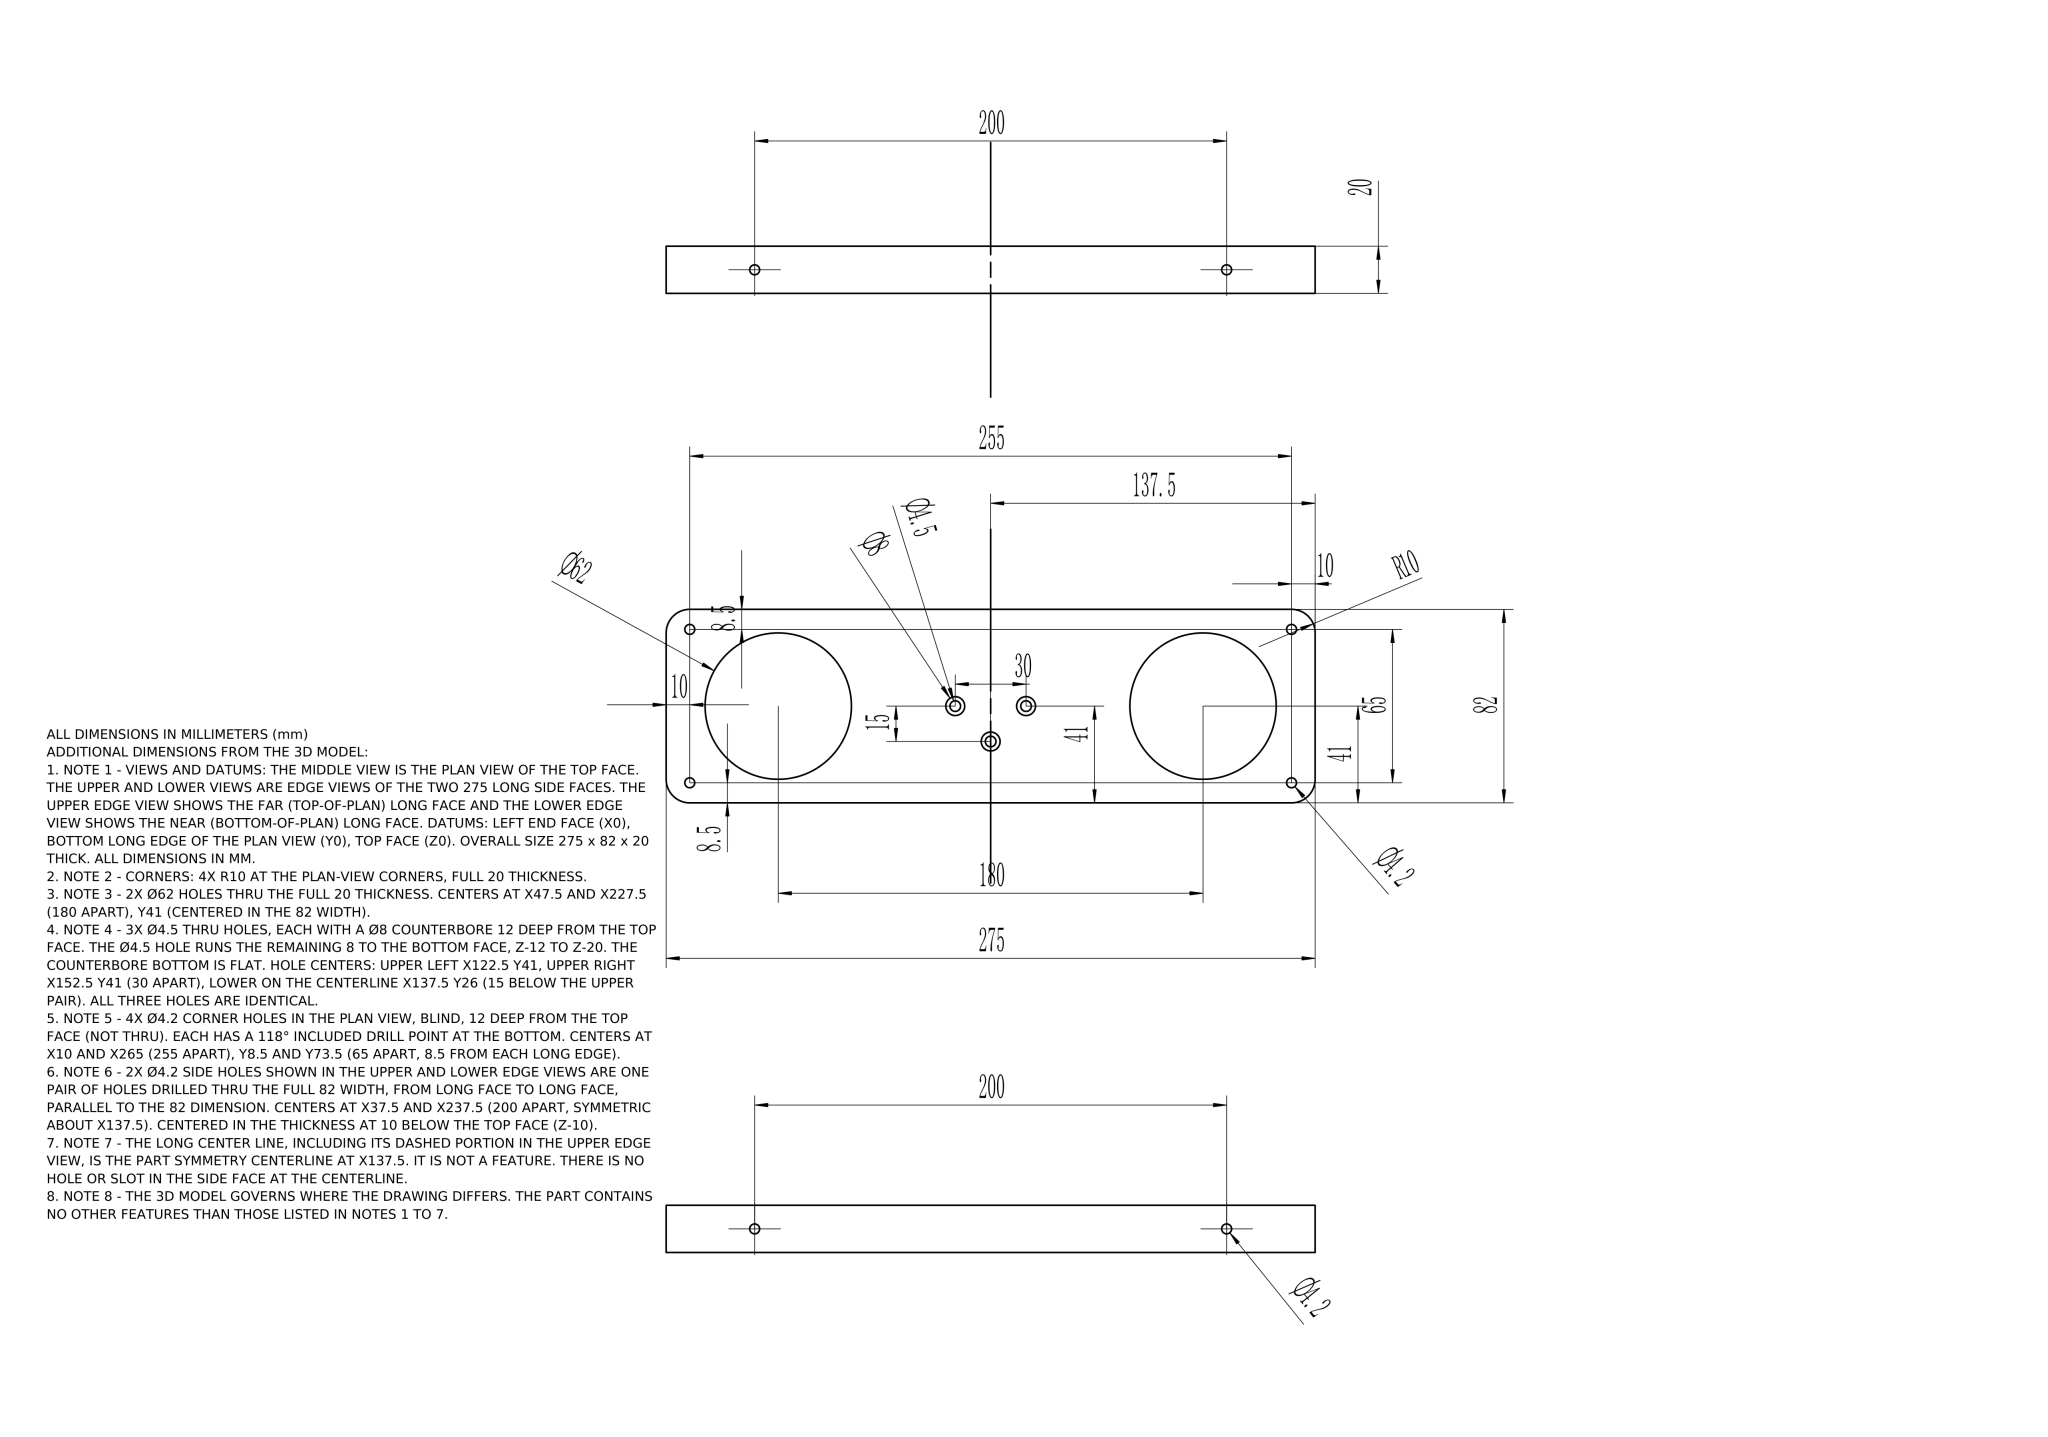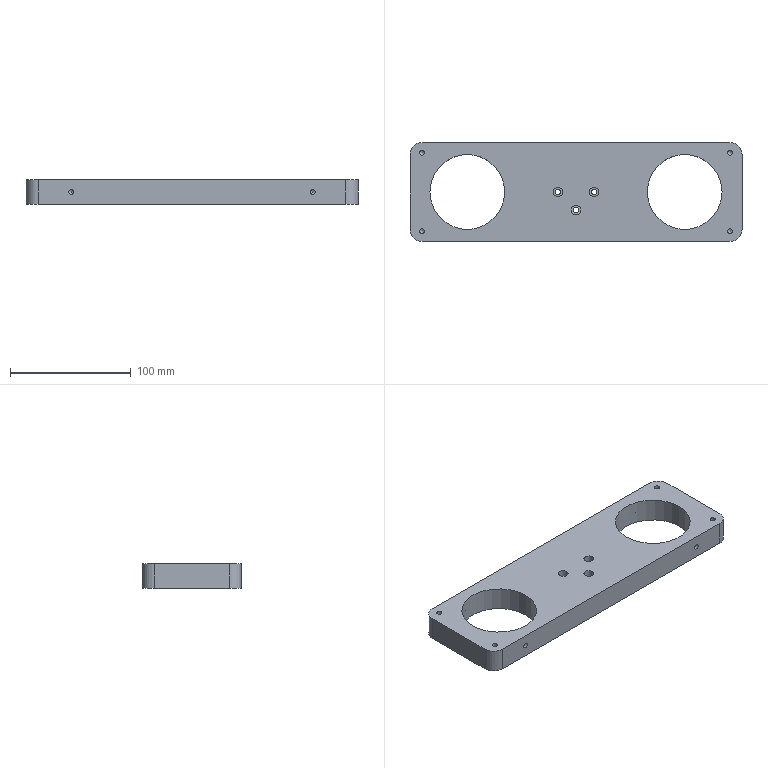Part | NX | mm | 1 solid | 37 faces | box 275 x 82 x 20 mm | volume 325063 mm3 | cylinder 20 | plane 9 | cone 8 | commonest cylinder face diameters 4.2 x8 20 x4 4.5 x3 8 x3 62 x2
STEP:
#1=CARTESIAN_POINT('',(0.,0.,0.));
#2=DIRECTION('',(0.,0.,1.));
#3=DIRECTION('',(1.,0.,0.));
#4=AXIS2_PLACEMENT_3D('',#1,#2,#3);
#5=(LENGTH_UNIT()NAMED_UNIT(*)SI_UNIT(.MILLI.,.METRE.));
#6=UNCERTAINTY_MEASURE_WITH_UNIT(LENGTH_MEASURE(0.00002),#5,'','');
#7=(NAMED_UNIT(*)PLANE_ANGLE_UNIT()SI_UNIT($,.RADIAN.));
#8=PLANE_ANGLE_MEASURE_WITH_UNIT(PLANE_ANGLE_MEASURE(0.01745),#7);
#9=DIMENSIONAL_EXPONENTS(0.,0.,0.,0.,0.,0.,0.);
#10=(CONVERSION_BASED_UNIT('',#8)NAMED_UNIT(#9)PLANE_ANGLE_UNIT());
#11=(NAMED_UNIT(*)SI_UNIT($,.STERADIAN.)SOLID_ANGLE_UNIT());
#12=(GEOMETRIC_REPRESENTATION_CONTEXT(3)GLOBAL_UNCERTAINTY_ASSIGNED_CONTEXT((#6))GLOBAL_UNIT_ASSIGNED_CONTEXT((#5,#10,#11))REPRESENTATION_CONTEXT('',''));
#13=SHAPE_REPRESENTATION('',(#4),#12);
#14=CARTESIAN_POINT('',(148.5,41.,0.));
#15=VERTEX_POINT('',#14);
#16=CARTESIAN_POINT('',(152.5,41.,0.));
#17=DIRECTION('',(0.,0.,-1.));
#18=DIRECTION('',(-1.,0.,0.));
#19=AXIS2_PLACEMENT_3D('',#16,#17,#18);
#20=CIRCLE('',#19,4.);
#21=EDGE_CURVE('',#15,#15,#20,.T.);
#22=ORIENTED_EDGE('',*,*,#21,.T.);
#23=EDGE_LOOP('',(#22));
#24=FACE_BOUND('',#23,.T.);
#25=CARTESIAN_POINT('',(133.5,26.,0.));
#26=VERTEX_POINT('',#25);
#27=CARTESIAN_POINT('',(137.5,26.,0.));
#28=DIRECTION('',(0.,0.,-1.));
#29=DIRECTION('',(-1.,0.,0.));
#30=AXIS2_PLACEMENT_3D('',#27,#28,#29);
#31=CIRCLE('',#30,4.);
#32=EDGE_CURVE('',#26,#26,#31,.T.);
#33=ORIENTED_EDGE('',*,*,#32,.T.);
#34=EDGE_LOOP('',(#33));
#35=FACE_BOUND('',#34,.T.);
#36=CARTESIAN_POINT('',(118.5,41.,0.));
#37=VERTEX_POINT('',#36);
#38=CARTESIAN_POINT('',(122.5,41.,0.));
#39=DIRECTION('',(0.,0.,-1.));
#40=DIRECTION('',(-1.,0.,0.));
#41=AXIS2_PLACEMENT_3D('',#38,#39,#40);
#42=CIRCLE('',#41,4.);
#43=EDGE_CURVE('',#37,#37,#42,.T.);
#44=ORIENTED_EDGE('',*,*,#43,.T.);
#45=EDGE_LOOP('',(#44));
#46=FACE_BOUND('',#45,.T.);
#47=CARTESIAN_POINT('',(262.9,73.5,0.));
#48=VERTEX_POINT('',#47);
#49=CARTESIAN_POINT('',(265.,73.5,0.));
#50=DIRECTION('',(0.,0.,-1.));
#51=DIRECTION('',(-1.,0.,0.));
#52=AXIS2_PLACEMENT_3D('',#49,#50,#51);
#53=CIRCLE('',#52,2.1);
#54=EDGE_CURVE('',#48,#48,#53,.T.);
#55=ORIENTED_EDGE('',*,*,#54,.T.);
#56=EDGE_LOOP('',(#55));
#57=FACE_BOUND('',#56,.T.);
#58=CARTESIAN_POINT('',(262.9,8.5,0.));
#59=VERTEX_POINT('',#58);
#60=CARTESIAN_POINT('',(265.,8.5,0.));
#61=DIRECTION('',(0.,0.,-1.));
#62=DIRECTION('',(-1.,0.,0.));
#63=AXIS2_PLACEMENT_3D('',#60,#61,#62);
#64=CIRCLE('',#63,2.1);
#65=EDGE_CURVE('',#59,#59,#64,.T.);
#66=ORIENTED_EDGE('',*,*,#65,.T.);
#67=EDGE_LOOP('',(#66));
#68=FACE_BOUND('',#67,.T.);
#69=CARTESIAN_POINT('',(7.9,73.5,0.));
#70=VERTEX_POINT('',#69);
#71=CARTESIAN_POINT('',(10.,73.5,0.));
#72=DIRECTION('',(0.,0.,-1.));
#73=DIRECTION('',(-1.,0.,0.));
#74=AXIS2_PLACEMENT_3D('',#71,#72,#73);
#75=CIRCLE('',#74,2.1);
#76=EDGE_CURVE('',#70,#70,#75,.T.);
#77=ORIENTED_EDGE('',*,*,#76,.T.);
#78=EDGE_LOOP('',(#77));
#79=FACE_BOUND('',#78,.T.);
#80=CARTESIAN_POINT('',(7.9,8.5,0.));
#81=VERTEX_POINT('',#80);
#82=CARTESIAN_POINT('',(10.,8.5,0.));
#83=DIRECTION('',(0.,0.,-1.));
#84=DIRECTION('',(-1.,0.,0.));
#85=AXIS2_PLACEMENT_3D('',#82,#83,#84);
#86=CIRCLE('',#85,2.1);
#87=EDGE_CURVE('',#81,#81,#86,.T.);
#88=ORIENTED_EDGE('',*,*,#87,.T.);
#89=EDGE_LOOP('',(#88));
#90=FACE_BOUND('',#89,.T.);
#91=CARTESIAN_POINT('',(196.5,41.,0.));
#92=VERTEX_POINT('',#91);
#93=CARTESIAN_POINT('',(227.5,41.,0.));
#94=DIRECTION('',(0.,0.,-1.));
#95=DIRECTION('',(-1.,0.,0.));
#96=AXIS2_PLACEMENT_3D('',#93,#94,#95);
#97=CIRCLE('',#96,31.);
#98=EDGE_CURVE('',#92,#92,#97,.T.);
#99=ORIENTED_EDGE('',*,*,#98,.T.);
#100=EDGE_LOOP('',(#99));
#101=FACE_BOUND('',#100,.T.);
#102=CARTESIAN_POINT('',(16.5,41.,0.));
#103=VERTEX_POINT('',#102);
#104=CARTESIAN_POINT('',(47.5,41.,0.));
#105=DIRECTION('',(0.,0.,-1.));
#106=DIRECTION('',(-1.,0.,0.));
#107=AXIS2_PLACEMENT_3D('',#104,#105,#106);
#108=CIRCLE('',#107,31.);
#109=EDGE_CURVE('',#103,#103,#108,.T.);
#110=ORIENTED_EDGE('',*,*,#109,.T.);
#111=EDGE_LOOP('',(#110));
#112=FACE_BOUND('',#111,.T.);
#113=CARTESIAN_POINT('',(275.,72.,0.));
#114=VERTEX_POINT('',#113);
#115=CARTESIAN_POINT('',(275.,10.,0.));
#116=VERTEX_POINT('',#115);
#117=CARTESIAN_POINT('',(275.,41.,0.));
#118=DIRECTION('',(0.,-1.,0.));
#119=VECTOR('',#118,1.);
#120=LINE('',#117,#119);
#121=EDGE_CURVE('',#114,#116,#120,.T.);
#122=ORIENTED_EDGE('',*,*,#121,.F.);
#123=CARTESIAN_POINT('',(265.,82.,0.));
#124=VERTEX_POINT('',#123);
#125=CARTESIAN_POINT('',(265.,72.,0.));
#126=DIRECTION('',(0.,0.,1.));
#127=DIRECTION('',(1.,0.,0.));
#128=AXIS2_PLACEMENT_3D('',#125,#126,#127);
#129=CIRCLE('',#128,10.);
#130=EDGE_CURVE('',#114,#124,#129,.T.);
#131=ORIENTED_EDGE('',*,*,#130,.T.);
#132=CARTESIAN_POINT('',(10.,82.,0.));
#133=VERTEX_POINT('',#132);
#134=CARTESIAN_POINT('',(137.5,82.,0.));
#135=DIRECTION('',(1.,0.,0.));
#136=VECTOR('',#135,1.);
#137=LINE('',#134,#136);
#138=EDGE_CURVE('',#133,#124,#137,.T.);
#139=ORIENTED_EDGE('',*,*,#138,.F.);
#140=CARTESIAN_POINT('',(0.,72.,0.));
#141=VERTEX_POINT('',#140);
#142=CARTESIAN_POINT('',(10.,72.,0.));
#143=DIRECTION('',(0.,0.,1.));
#144=DIRECTION('',(1.,0.,0.));
#145=AXIS2_PLACEMENT_3D('',#142,#143,#144);
#146=CIRCLE('',#145,10.);
#147=EDGE_CURVE('',#133,#141,#146,.T.);
#148=ORIENTED_EDGE('',*,*,#147,.T.);
#149=CARTESIAN_POINT('',(0.,10.,0.));
#150=VERTEX_POINT('',#149);
#151=CARTESIAN_POINT('',(0.,41.,0.));
#152=DIRECTION('',(0.,1.,0.));
#153=VECTOR('',#152,1.);
#154=LINE('',#151,#153);
#155=EDGE_CURVE('',#150,#141,#154,.T.);
#156=ORIENTED_EDGE('',*,*,#155,.F.);
#157=CARTESIAN_POINT('',(10.,0.,0.));
#158=VERTEX_POINT('',#157);
#159=CARTESIAN_POINT('',(10.,10.,0.));
#160=DIRECTION('',(0.,0.,1.));
#161=DIRECTION('',(1.,0.,0.));
#162=AXIS2_PLACEMENT_3D('',#159,#160,#161);
#163=CIRCLE('',#162,10.);
#164=EDGE_CURVE('',#150,#158,#163,.T.);
#165=ORIENTED_EDGE('',*,*,#164,.T.);
#166=CARTESIAN_POINT('',(265.,0.,0.));
#167=VERTEX_POINT('',#166);
#168=CARTESIAN_POINT('',(137.5,0.,0.));
#169=DIRECTION('',(-1.,0.,0.));
#170=VECTOR('',#169,1.);
#171=LINE('',#168,#170);
#172=EDGE_CURVE('',#167,#158,#171,.T.);
#173=ORIENTED_EDGE('',*,*,#172,.F.);
#174=CARTESIAN_POINT('',(265.,10.,0.));
#175=DIRECTION('',(0.,0.,1.));
#176=DIRECTION('',(1.,0.,0.));
#177=AXIS2_PLACEMENT_3D('',#174,#175,#176);
#178=CIRCLE('',#177,10.);
#179=EDGE_CURVE('',#167,#116,#178,.T.);
#180=ORIENTED_EDGE('',*,*,#179,.T.);
#181=EDGE_LOOP('',(#122,#131,#139,#148,#156,#165,#173,#180));
#182=FACE_BOUND('',#181,.T.);
#183=CARTESIAN_POINT('',(137.5,41.,0.));
#184=DIRECTION('',(0.,0.,1.));
#185=DIRECTION('',(1.,0.,0.));
#186=AXIS2_PLACEMENT_3D('',#183,#184,#185);
#187=PLANE('',#186);
#188=ADVANCED_FACE('',(#24,#35,#46,#57,#68,#79,#90,#101,#112,#182),#187,.T.);
#189=CARTESIAN_POINT('',(237.5,0.,-7.9));
#190=VERTEX_POINT('',#189);
#191=CARTESIAN_POINT('',(237.5,0.,-10.));
#192=DIRECTION('',(0.,1.,0.));
#193=DIRECTION('',(0.,0.,1.));
#194=AXIS2_PLACEMENT_3D('',#191,#192,#193);
#195=CIRCLE('',#194,2.1);
#196=EDGE_CURVE('',#190,#190,#195,.T.);
#197=ORIENTED_EDGE('',*,*,#196,.T.);
#198=EDGE_LOOP('',(#197));
#199=FACE_BOUND('',#198,.T.);
#200=CARTESIAN_POINT('',(37.5,0.,-7.9));
#201=VERTEX_POINT('',#200);
#202=CARTESIAN_POINT('',(37.5,0.,-10.));
#203=DIRECTION('',(0.,1.,0.));
#204=DIRECTION('',(0.,0.,1.));
#205=AXIS2_PLACEMENT_3D('',#202,#203,#204);
#206=CIRCLE('',#205,2.1);
#207=EDGE_CURVE('',#201,#201,#206,.T.);
#208=ORIENTED_EDGE('',*,*,#207,.T.);
#209=EDGE_LOOP('',(#208));
#210=FACE_BOUND('',#209,.T.);
#211=CARTESIAN_POINT('',(10.,0.,-20.));
#212=VERTEX_POINT('',#211);
#213=CARTESIAN_POINT('',(265.,0.,-20.));
#214=VERTEX_POINT('',#213);
#215=CARTESIAN_POINT('',(137.5,0.,-20.));
#216=DIRECTION('',(1.,0.,0.));
#217=VECTOR('',#216,1.);
#218=LINE('',#215,#217);
#219=EDGE_CURVE('',#212,#214,#218,.T.);
#220=ORIENTED_EDGE('',*,*,#219,.T.);
#221=CARTESIAN_POINT('',(265.,0.,-20.));
#222=DIRECTION('',(0.,0.,1.));
#223=VECTOR('',#222,1.);
#224=LINE('',#221,#223);
#225=EDGE_CURVE('',#214,#167,#224,.T.);
#226=ORIENTED_EDGE('',*,*,#225,.T.);
#227=ORIENTED_EDGE('',*,*,#172,.T.);
#228=CARTESIAN_POINT('',(10.,0.,-20.));
#229=DIRECTION('',(0.,0.,-1.));
#230=VECTOR('',#229,1.);
#231=LINE('',#228,#230);
#232=EDGE_CURVE('',#158,#212,#231,.T.);
#233=ORIENTED_EDGE('',*,*,#232,.T.);
#234=EDGE_LOOP('',(#220,#226,#227,#233));
#235=FACE_BOUND('',#234,.T.);
#236=CARTESIAN_POINT('',(137.5,0.,-20.));
#237=DIRECTION('',(0.,-1.,0.));
#238=DIRECTION('',(0.,0.,-1.));
#239=AXIS2_PLACEMENT_3D('',#236,#237,#238);
#240=PLANE('',#239);
#241=ADVANCED_FACE('',(#199,#210,#235),#240,.T.);
#242=ORIENTED_EDGE('',*,*,#155,.T.);
#243=CARTESIAN_POINT('',(0.,72.,-20.));
#244=VERTEX_POINT('',#243);
#245=CARTESIAN_POINT('',(0.,72.,-20.));
#246=DIRECTION('',(0.,0.,-1.));
#247=VECTOR('',#246,1.);
#248=LINE('',#245,#247);
#249=EDGE_CURVE('',#141,#244,#248,.T.);
#250=ORIENTED_EDGE('',*,*,#249,.T.);
#251=CARTESIAN_POINT('',(0.,10.,-20.));
#252=VERTEX_POINT('',#251);
#253=CARTESIAN_POINT('',(0.,41.,-20.));
#254=DIRECTION('',(0.,-1.,0.));
#255=VECTOR('',#254,1.);
#256=LINE('',#253,#255);
#257=EDGE_CURVE('',#244,#252,#256,.T.);
#258=ORIENTED_EDGE('',*,*,#257,.T.);
#259=CARTESIAN_POINT('',(0.,10.,-20.));
#260=DIRECTION('',(0.,0.,1.));
#261=VECTOR('',#260,1.);
#262=LINE('',#259,#261);
#263=EDGE_CURVE('',#252,#150,#262,.T.);
#264=ORIENTED_EDGE('',*,*,#263,.T.);
#265=EDGE_LOOP('',(#242,#250,#258,#264));
#266=FACE_OUTER_BOUND('',#265,.T.);
#267=CARTESIAN_POINT('',(0.,41.,-20.));
#268=DIRECTION('',(-1.,0.,0.));
#269=DIRECTION('',(0.,0.,1.));
#270=AXIS2_PLACEMENT_3D('',#267,#268,#269);
#271=PLANE('',#270);
#272=ADVANCED_FACE('',(#266),#271,.T.);
#273=CARTESIAN_POINT('',(237.5,82.,-12.1));
#274=VERTEX_POINT('',#273);
#275=CARTESIAN_POINT('',(237.5,82.,-10.));
#276=DIRECTION('',(0.,-1.,0.));
#277=DIRECTION('',(0.,0.,-1.));
#278=AXIS2_PLACEMENT_3D('',#275,#276,#277);
#279=CIRCLE('',#278,2.1);
#280=EDGE_CURVE('',#274,#274,#279,.T.);
#281=ORIENTED_EDGE('',*,*,#280,.T.);
#282=EDGE_LOOP('',(#281));
#283=FACE_BOUND('',#282,.T.);
#284=CARTESIAN_POINT('',(37.5,82.,-12.1));
#285=VERTEX_POINT('',#284);
#286=CARTESIAN_POINT('',(37.5,82.,-10.));
#287=DIRECTION('',(0.,-1.,0.));
#288=DIRECTION('',(0.,0.,-1.));
#289=AXIS2_PLACEMENT_3D('',#286,#287,#288);
#290=CIRCLE('',#289,2.1);
#291=EDGE_CURVE('',#285,#285,#290,.T.);
#292=ORIENTED_EDGE('',*,*,#291,.T.);
#293=EDGE_LOOP('',(#292));
#294=FACE_BOUND('',#293,.T.);
#295=ORIENTED_EDGE('',*,*,#138,.T.);
#296=CARTESIAN_POINT('',(265.,82.,-20.));
#297=VERTEX_POINT('',#296);
#298=CARTESIAN_POINT('',(265.,82.,-20.));
#299=DIRECTION('',(0.,0.,-1.));
#300=VECTOR('',#299,1.);
#301=LINE('',#298,#300);
#302=EDGE_CURVE('',#124,#297,#301,.T.);
#303=ORIENTED_EDGE('',*,*,#302,.T.);
#304=CARTESIAN_POINT('',(10.,82.,-20.));
#305=VERTEX_POINT('',#304);
#306=CARTESIAN_POINT('',(137.5,82.,-20.));
#307=DIRECTION('',(-1.,0.,0.));
#308=VECTOR('',#307,1.);
#309=LINE('',#306,#308);
#310=EDGE_CURVE('',#297,#305,#309,.T.);
#311=ORIENTED_EDGE('',*,*,#310,.T.);
#312=CARTESIAN_POINT('',(10.,82.,-20.));
#313=DIRECTION('',(0.,0.,1.));
#314=VECTOR('',#313,1.);
#315=LINE('',#312,#314);
#316=EDGE_CURVE('',#305,#133,#315,.T.);
#317=ORIENTED_EDGE('',*,*,#316,.T.);
#318=EDGE_LOOP('',(#295,#303,#311,#317));
#319=FACE_BOUND('',#318,.T.);
#320=CARTESIAN_POINT('',(137.5,82.,-20.));
#321=DIRECTION('',(0.,1.,0.));
#322=DIRECTION('',(0.,0.,1.));
#323=AXIS2_PLACEMENT_3D('',#320,#321,#322);
#324=PLANE('',#323);
#325=ADVANCED_FACE('',(#283,#294,#319),#324,.T.);
#326=CARTESIAN_POINT('',(150.25,41.,-20.));
#327=VERTEX_POINT('',#326);
#328=CARTESIAN_POINT('',(152.5,41.,-20.));
#329=DIRECTION('',(0.,0.,-1.));
#330=DIRECTION('',(-1.,0.,0.));
#331=AXIS2_PLACEMENT_3D('',#328,#329,#330);
#332=CIRCLE('',#331,2.25);
#333=EDGE_CURVE('',#327,#327,#332,.T.);
#334=ORIENTED_EDGE('',*,*,#333,.F.);
#335=EDGE_LOOP('',(#334));
#336=FACE_BOUND('',#335,.T.);
#337=CARTESIAN_POINT('',(135.25,26.,-20.));
#338=VERTEX_POINT('',#337);
#339=CARTESIAN_POINT('',(137.5,26.,-20.));
#340=DIRECTION('',(0.,0.,-1.));
#341=DIRECTION('',(-1.,0.,0.));
#342=AXIS2_PLACEMENT_3D('',#339,#340,#341);
#343=CIRCLE('',#342,2.25);
#344=EDGE_CURVE('',#338,#338,#343,.T.);
#345=ORIENTED_EDGE('',*,*,#344,.F.);
#346=EDGE_LOOP('',(#345));
#347=FACE_BOUND('',#346,.T.);
#348=CARTESIAN_POINT('',(120.25,41.,-20.));
#349=VERTEX_POINT('',#348);
#350=CARTESIAN_POINT('',(122.5,41.,-20.));
#351=DIRECTION('',(0.,0.,-1.));
#352=DIRECTION('',(-1.,0.,0.));
#353=AXIS2_PLACEMENT_3D('',#350,#351,#352);
#354=CIRCLE('',#353,2.25);
#355=EDGE_CURVE('',#349,#349,#354,.T.);
#356=ORIENTED_EDGE('',*,*,#355,.F.);
#357=EDGE_LOOP('',(#356));
#358=FACE_BOUND('',#357,.T.);
#359=CARTESIAN_POINT('',(196.5,41.,-20.));
#360=VERTEX_POINT('',#359);
#361=CARTESIAN_POINT('',(227.5,41.,-20.));
#362=DIRECTION('',(0.,0.,-1.));
#363=DIRECTION('',(-1.,0.,0.));
#364=AXIS2_PLACEMENT_3D('',#361,#362,#363);
#365=CIRCLE('',#364,31.);
#366=EDGE_CURVE('',#360,#360,#365,.T.);
#367=ORIENTED_EDGE('',*,*,#366,.F.);
#368=EDGE_LOOP('',(#367));
#369=FACE_BOUND('',#368,.T.);
#370=CARTESIAN_POINT('',(16.5,41.,-20.));
#371=VERTEX_POINT('',#370);
#372=CARTESIAN_POINT('',(47.5,41.,-20.));
#373=DIRECTION('',(0.,0.,-1.));
#374=DIRECTION('',(-1.,0.,0.));
#375=AXIS2_PLACEMENT_3D('',#372,#373,#374);
#376=CIRCLE('',#375,31.);
#377=EDGE_CURVE('',#371,#371,#376,.T.);
#378=ORIENTED_EDGE('',*,*,#377,.F.);
#379=EDGE_LOOP('',(#378));
#380=FACE_BOUND('',#379,.T.);
#381=ORIENTED_EDGE('',*,*,#310,.F.);
#382=CARTESIAN_POINT('',(275.,72.,-20.));
#383=VERTEX_POINT('',#382);
#384=CARTESIAN_POINT('',(265.,72.,-20.));
#385=DIRECTION('',(0.,0.,-1.));
#386=DIRECTION('',(-1.,0.,0.));
#387=AXIS2_PLACEMENT_3D('',#384,#385,#386);
#388=CIRCLE('',#387,10.);
#389=EDGE_CURVE('',#297,#383,#388,.T.);
#390=ORIENTED_EDGE('',*,*,#389,.T.);
#391=CARTESIAN_POINT('',(275.,10.,-20.));
#392=VERTEX_POINT('',#391);
#393=CARTESIAN_POINT('',(275.,41.,-20.));
#394=DIRECTION('',(0.,1.,0.));
#395=VECTOR('',#394,1.);
#396=LINE('',#393,#395);
#397=EDGE_CURVE('',#392,#383,#396,.T.);
#398=ORIENTED_EDGE('',*,*,#397,.F.);
#399=CARTESIAN_POINT('',(265.,10.,-20.));
#400=DIRECTION('',(0.,0.,-1.));
#401=DIRECTION('',(-1.,0.,0.));
#402=AXIS2_PLACEMENT_3D('',#399,#400,#401);
#403=CIRCLE('',#402,10.);
#404=EDGE_CURVE('',#392,#214,#403,.T.);
#405=ORIENTED_EDGE('',*,*,#404,.T.);
#406=ORIENTED_EDGE('',*,*,#219,.F.);
#407=CARTESIAN_POINT('',(10.,10.,-20.));
#408=DIRECTION('',(0.,0.,-1.));
#409=DIRECTION('',(-1.,0.,0.));
#410=AXIS2_PLACEMENT_3D('',#407,#408,#409);
#411=CIRCLE('',#410,10.);
#412=EDGE_CURVE('',#212,#252,#411,.T.);
#413=ORIENTED_EDGE('',*,*,#412,.T.);
#414=ORIENTED_EDGE('',*,*,#257,.F.);
#415=CARTESIAN_POINT('',(10.,72.,-20.));
#416=DIRECTION('',(0.,0.,-1.));
#417=DIRECTION('',(-1.,0.,0.));
#418=AXIS2_PLACEMENT_3D('',#415,#416,#417);
#419=CIRCLE('',#418,10.);
#420=EDGE_CURVE('',#244,#305,#419,.T.);
#421=ORIENTED_EDGE('',*,*,#420,.T.);
#422=EDGE_LOOP('',(#381,#390,#398,#405,#406,#413,#414,#421));
#423=FACE_BOUND('',#422,.T.);
#424=CARTESIAN_POINT('',(137.5,41.,-20.));
#425=DIRECTION('',(0.,0.,-1.));
#426=DIRECTION('',(-1.,0.,0.));
#427=AXIS2_PLACEMENT_3D('',#424,#425,#426);
#428=PLANE('',#427);
#429=ADVANCED_FACE('',(#336,#347,#358,#369,#380,#423),#428,.T.);
#430=ORIENTED_EDGE('',*,*,#397,.T.);
#431=CARTESIAN_POINT('',(275.,72.,-20.));
#432=DIRECTION('',(0.,0.,1.));
#433=VECTOR('',#432,1.);
#434=LINE('',#431,#433);
#435=EDGE_CURVE('',#383,#114,#434,.T.);
#436=ORIENTED_EDGE('',*,*,#435,.T.);
#437=ORIENTED_EDGE('',*,*,#121,.T.);
#438=CARTESIAN_POINT('',(275.,10.,-20.));
#439=DIRECTION('',(0.,0.,-1.));
#440=VECTOR('',#439,1.);
#441=LINE('',#438,#440);
#442=EDGE_CURVE('',#116,#392,#441,.T.);
#443=ORIENTED_EDGE('',*,*,#442,.T.);
#444=EDGE_LOOP('',(#430,#436,#437,#443));
#445=FACE_OUTER_BOUND('',#444,.T.);
#446=CARTESIAN_POINT('',(275.,41.,-20.));
#447=DIRECTION('',(1.,0.,0.));
#448=DIRECTION('',(0.,0.,-1.));
#449=AXIS2_PLACEMENT_3D('',#446,#447,#448);
#450=PLANE('',#449);
#451=ADVANCED_FACE('',(#445),#450,.T.);
#452=ORIENTED_EDGE('',*,*,#389,.F.);
#453=ORIENTED_EDGE('',*,*,#302,.F.);
#454=ORIENTED_EDGE('',*,*,#130,.F.);
#455=ORIENTED_EDGE('',*,*,#435,.F.);
#456=EDGE_LOOP('',(#452,#453,#454,#455));
#457=FACE_OUTER_BOUND('',#456,.T.);
#458=CARTESIAN_POINT('',(265.,72.,-20.));
#459=DIRECTION('',(0.,0.,1.));
#460=DIRECTION('',(1.,0.,0.));
#461=AXIS2_PLACEMENT_3D('',#458,#459,#460);
#462=CYLINDRICAL_SURFACE('',#461,10.);
#463=ADVANCED_FACE('',(#457),#462,.T.);
#464=ORIENTED_EDGE('',*,*,#404,.F.);
#465=ORIENTED_EDGE('',*,*,#442,.F.);
#466=ORIENTED_EDGE('',*,*,#179,.F.);
#467=ORIENTED_EDGE('',*,*,#225,.F.);
#468=EDGE_LOOP('',(#464,#465,#466,#467));
#469=FACE_OUTER_BOUND('',#468,.T.);
#470=CARTESIAN_POINT('',(265.,10.,-20.));
#471=DIRECTION('',(0.,0.,1.));
#472=DIRECTION('',(1.,0.,0.));
#473=AXIS2_PLACEMENT_3D('',#470,#471,#472);
#474=CYLINDRICAL_SURFACE('',#473,10.);
#475=ADVANCED_FACE('',(#469),#474,.T.);
#476=ORIENTED_EDGE('',*,*,#420,.F.);
#477=ORIENTED_EDGE('',*,*,#249,.F.);
#478=ORIENTED_EDGE('',*,*,#147,.F.);
#479=ORIENTED_EDGE('',*,*,#316,.F.);
#480=EDGE_LOOP('',(#476,#477,#478,#479));
#481=FACE_OUTER_BOUND('',#480,.T.);
#482=CARTESIAN_POINT('',(10.,72.,-20.));
#483=DIRECTION('',(0.,0.,1.));
#484=DIRECTION('',(1.,0.,0.));
#485=AXIS2_PLACEMENT_3D('',#482,#483,#484);
#486=CYLINDRICAL_SURFACE('',#485,10.);
#487=ADVANCED_FACE('',(#481),#486,.T.);
#488=ORIENTED_EDGE('',*,*,#412,.F.);
#489=ORIENTED_EDGE('',*,*,#232,.F.);
#490=ORIENTED_EDGE('',*,*,#164,.F.);
#491=ORIENTED_EDGE('',*,*,#263,.F.);
#492=EDGE_LOOP('',(#488,#489,#490,#491));
#493=FACE_OUTER_BOUND('',#492,.T.);
#494=CARTESIAN_POINT('',(10.,10.,-20.));
#495=DIRECTION('',(0.,0.,1.));
#496=DIRECTION('',(1.,0.,0.));
#497=AXIS2_PLACEMENT_3D('',#494,#495,#496);
#498=CYLINDRICAL_SURFACE('',#497,10.);
#499=ADVANCED_FACE('',(#493),#498,.T.);
#500=ORIENTED_EDGE('',*,*,#377,.T.);
#501=EDGE_LOOP('',(#500));
#502=FACE_BOUND('',#501,.T.);
#503=ORIENTED_EDGE('',*,*,#109,.F.);
#504=EDGE_LOOP('',(#503));
#505=FACE_BOUND('',#504,.T.);
#506=CARTESIAN_POINT('',(47.5,41.,0.));
#507=DIRECTION('',(0.,0.,-1.));
#508=DIRECTION('',(-1.,0.,0.));
#509=AXIS2_PLACEMENT_3D('',#506,#507,#508);
#510=CYLINDRICAL_SURFACE('',#509,31.);
#511=ADVANCED_FACE('',(#502,#505),#510,.F.);
#512=ORIENTED_EDGE('',*,*,#366,.T.);
#513=EDGE_LOOP('',(#512));
#514=FACE_BOUND('',#513,.T.);
#515=ORIENTED_EDGE('',*,*,#98,.F.);
#516=EDGE_LOOP('',(#515));
#517=FACE_BOUND('',#516,.T.);
#518=CARTESIAN_POINT('',(227.5,41.,0.));
#519=DIRECTION('',(0.,0.,-1.));
#520=DIRECTION('',(-1.,0.,0.));
#521=AXIS2_PLACEMENT_3D('',#518,#519,#520);
#522=CYLINDRICAL_SURFACE('',#521,31.);
#523=ADVANCED_FACE('',(#514,#517),#522,.F.);
#524=CARTESIAN_POINT('',(7.9,8.5,-12.));
#525=VERTEX_POINT('',#524);
#526=CARTESIAN_POINT('',(10.,8.5,-12.));
#527=DIRECTION('',(0.,0.,1.));
#528=DIRECTION('',(-1.,0.,0.));
#529=AXIS2_PLACEMENT_3D('',#526,#527,#528);
#530=CIRCLE('',#529,2.1);
#531=EDGE_CURVE('',#525,#525,#530,.T.);
#532=ORIENTED_EDGE('',*,*,#531,.T.);
#533=EDGE_LOOP('',(#532));
#534=FACE_BOUND('',#533,.T.);
#535=CARTESIAN_POINT('',(10.,8.5,-13.262));
#536=VERTEX_POINT('',#535);
#537=VERTEX_LOOP('',#536);
#538=FACE_BOUND('',#537,.T.);
#539=CARTESIAN_POINT('',(10.,8.5,-12.));
#540=DIRECTION('',(0.,0.,1.));
#541=DIRECTION('',(1.,0.,-0.));
#542=AXIS2_PLACEMENT_3D('',#539,#540,#541);
#543=CONICAL_SURFACE('',#542,2.1,59.);
#544=ADVANCED_FACE('',(#534,#538),#543,.F.);
#545=ORIENTED_EDGE('',*,*,#531,.F.);
#546=EDGE_LOOP('',(#545));
#547=FACE_BOUND('',#546,.T.);
#548=ORIENTED_EDGE('',*,*,#87,.F.);
#549=EDGE_LOOP('',(#548));
#550=FACE_BOUND('',#549,.T.);
#551=CARTESIAN_POINT('',(10.,8.5,0.));
#552=DIRECTION('',(0.,0.,-1.));
#553=DIRECTION('',(-1.,0.,0.));
#554=AXIS2_PLACEMENT_3D('',#551,#552,#553);
#555=CYLINDRICAL_SURFACE('',#554,2.1);
#556=ADVANCED_FACE('',(#547,#550),#555,.F.);
#557=CARTESIAN_POINT('',(7.9,73.5,-12.));
#558=VERTEX_POINT('',#557);
#559=CARTESIAN_POINT('',(10.,73.5,-12.));
#560=DIRECTION('',(0.,0.,1.));
#561=DIRECTION('',(-1.,0.,0.));
#562=AXIS2_PLACEMENT_3D('',#559,#560,#561);
#563=CIRCLE('',#562,2.1);
#564=EDGE_CURVE('',#558,#558,#563,.T.);
#565=ORIENTED_EDGE('',*,*,#564,.T.);
#566=EDGE_LOOP('',(#565));
#567=FACE_BOUND('',#566,.T.);
#568=CARTESIAN_POINT('',(10.,73.5,-13.262));
#569=VERTEX_POINT('',#568);
#570=VERTEX_LOOP('',#569);
#571=FACE_BOUND('',#570,.T.);
#572=CARTESIAN_POINT('',(10.,73.5,-12.));
#573=DIRECTION('',(0.,0.,1.));
#574=DIRECTION('',(1.,0.,-0.));
#575=AXIS2_PLACEMENT_3D('',#572,#573,#574);
#576=CONICAL_SURFACE('',#575,2.1,59.);
#577=ADVANCED_FACE('',(#567,#571),#576,.F.);
#578=ORIENTED_EDGE('',*,*,#564,.F.);
#579=EDGE_LOOP('',(#578));
#580=FACE_BOUND('',#579,.T.);
#581=ORIENTED_EDGE('',*,*,#76,.F.);
#582=EDGE_LOOP('',(#581));
#583=FACE_BOUND('',#582,.T.);
#584=CARTESIAN_POINT('',(10.,73.5,0.));
#585=DIRECTION('',(0.,0.,-1.));
#586=DIRECTION('',(-1.,0.,0.));
#587=AXIS2_PLACEMENT_3D('',#584,#585,#586);
#588=CYLINDRICAL_SURFACE('',#587,2.1);
#589=ADVANCED_FACE('',(#580,#583),#588,.F.);
#590=CARTESIAN_POINT('',(262.9,8.5,-12.));
#591=VERTEX_POINT('',#590);
#592=CARTESIAN_POINT('',(265.,8.5,-12.));
#593=DIRECTION('',(0.,0.,1.));
#594=DIRECTION('',(-1.,0.,0.));
#595=AXIS2_PLACEMENT_3D('',#592,#593,#594);
#596=CIRCLE('',#595,2.1);
#597=EDGE_CURVE('',#591,#591,#596,.T.);
#598=ORIENTED_EDGE('',*,*,#597,.T.);
#599=EDGE_LOOP('',(#598));
#600=FACE_BOUND('',#599,.T.);
#601=CARTESIAN_POINT('',(265.,8.5,-13.262));
#602=VERTEX_POINT('',#601);
#603=VERTEX_LOOP('',#602);
#604=FACE_BOUND('',#603,.T.);
#605=CARTESIAN_POINT('',(265.,8.5,-12.));
#606=DIRECTION('',(0.,0.,1.));
#607=DIRECTION('',(1.,0.,-0.));
#608=AXIS2_PLACEMENT_3D('',#605,#606,#607);
#609=CONICAL_SURFACE('',#608,2.1,59.);
#610=ADVANCED_FACE('',(#600,#604),#609,.F.);
#611=ORIENTED_EDGE('',*,*,#597,.F.);
#612=EDGE_LOOP('',(#611));
#613=FACE_BOUND('',#612,.T.);
#614=ORIENTED_EDGE('',*,*,#65,.F.);
#615=EDGE_LOOP('',(#614));
#616=FACE_BOUND('',#615,.T.);
#617=CARTESIAN_POINT('',(265.,8.5,0.));
#618=DIRECTION('',(0.,0.,-1.));
#619=DIRECTION('',(-1.,0.,0.));
#620=AXIS2_PLACEMENT_3D('',#617,#618,#619);
#621=CYLINDRICAL_SURFACE('',#620,2.1);
#622=ADVANCED_FACE('',(#613,#616),#621,.F.);
#623=CARTESIAN_POINT('',(262.9,73.5,-12.));
#624=VERTEX_POINT('',#623);
#625=CARTESIAN_POINT('',(265.,73.5,-12.));
#626=DIRECTION('',(0.,0.,1.));
#627=DIRECTION('',(-1.,0.,0.));
#628=AXIS2_PLACEMENT_3D('',#625,#626,#627);
#629=CIRCLE('',#628,2.1);
#630=EDGE_CURVE('',#624,#624,#629,.T.);
#631=ORIENTED_EDGE('',*,*,#630,.T.);
#632=EDGE_LOOP('',(#631));
#633=FACE_BOUND('',#632,.T.);
#634=CARTESIAN_POINT('',(265.,73.5,-13.262));
#635=VERTEX_POINT('',#634);
#636=VERTEX_LOOP('',#635);
#637=FACE_BOUND('',#636,.T.);
#638=CARTESIAN_POINT('',(265.,73.5,-12.));
#639=DIRECTION('',(0.,0.,1.));
#640=DIRECTION('',(1.,0.,-0.));
#641=AXIS2_PLACEMENT_3D('',#638,#639,#640);
#642=CONICAL_SURFACE('',#641,2.1,59.);
#643=ADVANCED_FACE('',(#633,#637),#642,.F.);
#644=ORIENTED_EDGE('',*,*,#630,.F.);
#645=EDGE_LOOP('',(#644));
#646=FACE_BOUND('',#645,.T.);
#647=ORIENTED_EDGE('',*,*,#54,.F.);
#648=EDGE_LOOP('',(#647));
#649=FACE_BOUND('',#648,.T.);
#650=CARTESIAN_POINT('',(265.,73.5,0.));
#651=DIRECTION('',(0.,0.,-1.));
#652=DIRECTION('',(-1.,0.,0.));
#653=AXIS2_PLACEMENT_3D('',#650,#651,#652);
#654=CYLINDRICAL_SURFACE('',#653,2.1);
#655=ADVANCED_FACE('',(#646,#649),#654,.F.);
#656=ORIENTED_EDGE('',*,*,#355,.T.);
#657=EDGE_LOOP('',(#656));
#658=FACE_BOUND('',#657,.T.);
#659=CARTESIAN_POINT('',(120.25,41.,-12.));
#660=VERTEX_POINT('',#659);
#661=CARTESIAN_POINT('',(122.5,41.,-12.));
#662=DIRECTION('',(0.,0.,1.));
#663=DIRECTION('',(-1.,0.,0.));
#664=AXIS2_PLACEMENT_3D('',#661,#662,#663);
#665=CIRCLE('',#664,2.25);
#666=EDGE_CURVE('',#660,#660,#665,.T.);
#667=ORIENTED_EDGE('',*,*,#666,.T.);
#668=EDGE_LOOP('',(#667));
#669=FACE_BOUND('',#668,.T.);
#670=CARTESIAN_POINT('',(122.5,41.,-50.));
#671=DIRECTION('',(0.,0.,-1.));
#672=DIRECTION('',(-1.,0.,0.));
#673=AXIS2_PLACEMENT_3D('',#670,#671,#672);
#674=CYLINDRICAL_SURFACE('',#673,2.25);
#675=ADVANCED_FACE('',(#658,#669),#674,.F.);
#676=ORIENTED_EDGE('',*,*,#666,.F.);
#677=EDGE_LOOP('',(#676));
#678=FACE_BOUND('',#677,.T.);
#679=CARTESIAN_POINT('',(118.5,41.,-12.));
#680=VERTEX_POINT('',#679);
#681=CARTESIAN_POINT('',(122.5,41.,-12.));
#682=DIRECTION('',(0.,0.,1.));
#683=DIRECTION('',(-1.,0.,0.));
#684=AXIS2_PLACEMENT_3D('',#681,#682,#683);
#685=CIRCLE('',#684,4.);
#686=EDGE_CURVE('',#680,#680,#685,.T.);
#687=ORIENTED_EDGE('',*,*,#686,.T.);
#688=EDGE_LOOP('',(#687));
#689=FACE_BOUND('',#688,.T.);
#690=CARTESIAN_POINT('',(122.5,41.,-12.));
#691=DIRECTION('',(0.,0.,-1.));
#692=DIRECTION('',(-1.,0.,0.));
#693=AXIS2_PLACEMENT_3D('',#690,#691,#692);
#694=PLANE('',#693);
#695=ADVANCED_FACE('',(#678,#689),#694,.F.);
#696=ORIENTED_EDGE('',*,*,#686,.F.);
#697=EDGE_LOOP('',(#696));
#698=FACE_BOUND('',#697,.T.);
#699=ORIENTED_EDGE('',*,*,#43,.F.);
#700=EDGE_LOOP('',(#699));
#701=FACE_BOUND('',#700,.T.);
#702=CARTESIAN_POINT('',(122.5,41.,0.));
#703=DIRECTION('',(0.,0.,-1.));
#704=DIRECTION('',(-1.,0.,0.));
#705=AXIS2_PLACEMENT_3D('',#702,#703,#704);
#706=CYLINDRICAL_SURFACE('',#705,4.);
#707=ADVANCED_FACE('',(#698,#701),#706,.F.);
#708=ORIENTED_EDGE('',*,*,#344,.T.);
#709=EDGE_LOOP('',(#708));
#710=FACE_BOUND('',#709,.T.);
#711=CARTESIAN_POINT('',(135.25,26.,-12.));
#712=VERTEX_POINT('',#711);
#713=CARTESIAN_POINT('',(137.5,26.,-12.));
#714=DIRECTION('',(0.,0.,1.));
#715=DIRECTION('',(-1.,0.,0.));
#716=AXIS2_PLACEMENT_3D('',#713,#714,#715);
#717=CIRCLE('',#716,2.25);
#718=EDGE_CURVE('',#712,#712,#717,.T.);
#719=ORIENTED_EDGE('',*,*,#718,.T.);
#720=EDGE_LOOP('',(#719));
#721=FACE_BOUND('',#720,.T.);
#722=CARTESIAN_POINT('',(137.5,26.,-50.));
#723=DIRECTION('',(0.,0.,-1.));
#724=DIRECTION('',(-1.,0.,0.));
#725=AXIS2_PLACEMENT_3D('',#722,#723,#724);
#726=CYLINDRICAL_SURFACE('',#725,2.25);
#727=ADVANCED_FACE('',(#710,#721),#726,.F.);
#728=ORIENTED_EDGE('',*,*,#718,.F.);
#729=EDGE_LOOP('',(#728));
#730=FACE_BOUND('',#729,.T.);
#731=CARTESIAN_POINT('',(133.5,26.,-12.));
#732=VERTEX_POINT('',#731);
#733=CARTESIAN_POINT('',(137.5,26.,-12.));
#734=DIRECTION('',(0.,0.,1.));
#735=DIRECTION('',(-1.,0.,0.));
#736=AXIS2_PLACEMENT_3D('',#733,#734,#735);
#737=CIRCLE('',#736,4.);
#738=EDGE_CURVE('',#732,#732,#737,.T.);
#739=ORIENTED_EDGE('',*,*,#738,.T.);
#740=EDGE_LOOP('',(#739));
#741=FACE_BOUND('',#740,.T.);
#742=CARTESIAN_POINT('',(137.5,26.,-12.));
#743=DIRECTION('',(0.,0.,-1.));
#744=DIRECTION('',(-1.,0.,0.));
#745=AXIS2_PLACEMENT_3D('',#742,#743,#744);
#746=PLANE('',#745);
#747=ADVANCED_FACE('',(#730,#741),#746,.F.);
#748=ORIENTED_EDGE('',*,*,#738,.F.);
#749=EDGE_LOOP('',(#748));
#750=FACE_BOUND('',#749,.T.);
#751=ORIENTED_EDGE('',*,*,#32,.F.);
#752=EDGE_LOOP('',(#751));
#753=FACE_BOUND('',#752,.T.);
#754=CARTESIAN_POINT('',(137.5,26.,0.));
#755=DIRECTION('',(0.,0.,-1.));
#756=DIRECTION('',(-1.,0.,0.));
#757=AXIS2_PLACEMENT_3D('',#754,#755,#756);
#758=CYLINDRICAL_SURFACE('',#757,4.);
#759=ADVANCED_FACE('',(#750,#753),#758,.F.);
#760=ORIENTED_EDGE('',*,*,#333,.T.);
#761=EDGE_LOOP('',(#760));
#762=FACE_BOUND('',#761,.T.);
#763=CARTESIAN_POINT('',(150.25,41.,-12.));
#764=VERTEX_POINT('',#763);
#765=CARTESIAN_POINT('',(152.5,41.,-12.));
#766=DIRECTION('',(0.,0.,1.));
#767=DIRECTION('',(-1.,0.,0.));
#768=AXIS2_PLACEMENT_3D('',#765,#766,#767);
#769=CIRCLE('',#768,2.25);
#770=EDGE_CURVE('',#764,#764,#769,.T.);
#771=ORIENTED_EDGE('',*,*,#770,.T.);
#772=EDGE_LOOP('',(#771));
#773=FACE_BOUND('',#772,.T.);
#774=CARTESIAN_POINT('',(152.5,41.,-50.));
#775=DIRECTION('',(0.,0.,-1.));
#776=DIRECTION('',(-1.,0.,0.));
#777=AXIS2_PLACEMENT_3D('',#774,#775,#776);
#778=CYLINDRICAL_SURFACE('',#777,2.25);
#779=ADVANCED_FACE('',(#762,#773),#778,.F.);
#780=ORIENTED_EDGE('',*,*,#770,.F.);
#781=EDGE_LOOP('',(#780));
#782=FACE_BOUND('',#781,.T.);
#783=CARTESIAN_POINT('',(148.5,41.,-12.));
#784=VERTEX_POINT('',#783);
#785=CARTESIAN_POINT('',(152.5,41.,-12.));
#786=DIRECTION('',(0.,0.,1.));
#787=DIRECTION('',(-1.,0.,0.));
#788=AXIS2_PLACEMENT_3D('',#785,#786,#787);
#789=CIRCLE('',#788,4.);
#790=EDGE_CURVE('',#784,#784,#789,.T.);
#791=ORIENTED_EDGE('',*,*,#790,.T.);
#792=EDGE_LOOP('',(#791));
#793=FACE_BOUND('',#792,.T.);
#794=CARTESIAN_POINT('',(152.5,41.,-12.));
#795=DIRECTION('',(0.,0.,-1.));
#796=DIRECTION('',(-1.,0.,0.));
#797=AXIS2_PLACEMENT_3D('',#794,#795,#796);
#798=PLANE('',#797);
#799=ADVANCED_FACE('',(#782,#793),#798,.F.);
#800=ORIENTED_EDGE('',*,*,#790,.F.);
#801=EDGE_LOOP('',(#800));
#802=FACE_BOUND('',#801,.T.);
#803=ORIENTED_EDGE('',*,*,#21,.F.);
#804=EDGE_LOOP('',(#803));
#805=FACE_BOUND('',#804,.T.);
#806=CARTESIAN_POINT('',(152.5,41.,0.));
#807=DIRECTION('',(0.,0.,-1.));
#808=DIRECTION('',(-1.,0.,0.));
#809=AXIS2_PLACEMENT_3D('',#806,#807,#808);
#810=CYLINDRICAL_SURFACE('',#809,4.);
#811=ADVANCED_FACE('',(#802,#805),#810,.F.);
#812=CARTESIAN_POINT('',(37.5,10.,-7.9));
#813=VERTEX_POINT('',#812);
#814=CARTESIAN_POINT('',(37.5,10.,-10.));
#815=DIRECTION('',(0.,-1.,0.));
#816=DIRECTION('',(0.,0.,1.));
#817=AXIS2_PLACEMENT_3D('',#814,#815,#816);
#818=CIRCLE('',#817,2.1);
#819=EDGE_CURVE('',#813,#813,#818,.T.);
#820=ORIENTED_EDGE('',*,*,#819,.T.);
#821=EDGE_LOOP('',(#820));
#822=FACE_BOUND('',#821,.T.);
#823=CARTESIAN_POINT('',(37.5,11.262,-10.));
#824=VERTEX_POINT('',#823);
#825=VERTEX_LOOP('',#824);
#826=FACE_BOUND('',#825,.T.);
#827=CARTESIAN_POINT('',(37.5,10.,-10.));
#828=DIRECTION('',(0.,-1.,0.));
#829=DIRECTION('',(0.,0.,-1.));
#830=AXIS2_PLACEMENT_3D('',#827,#828,#829);
#831=CONICAL_SURFACE('',#830,2.1,59.);
#832=ADVANCED_FACE('',(#822,#826),#831,.F.);
#833=ORIENTED_EDGE('',*,*,#819,.F.);
#834=EDGE_LOOP('',(#833));
#835=FACE_BOUND('',#834,.T.);
#836=ORIENTED_EDGE('',*,*,#207,.F.);
#837=EDGE_LOOP('',(#836));
#838=FACE_BOUND('',#837,.T.);
#839=CARTESIAN_POINT('',(37.5,0.,-10.));
#840=DIRECTION('',(0.,1.,0.));
#841=DIRECTION('',(0.,0.,1.));
#842=AXIS2_PLACEMENT_3D('',#839,#840,#841);
#843=CYLINDRICAL_SURFACE('',#842,2.1);
#844=ADVANCED_FACE('',(#835,#838),#843,.F.);
#845=CARTESIAN_POINT('',(237.5,10.,-7.9));
#846=VERTEX_POINT('',#845);
#847=CARTESIAN_POINT('',(237.5,10.,-10.));
#848=DIRECTION('',(0.,-1.,0.));
#849=DIRECTION('',(0.,0.,1.));
#850=AXIS2_PLACEMENT_3D('',#847,#848,#849);
#851=CIRCLE('',#850,2.1);
#852=EDGE_CURVE('',#846,#846,#851,.T.);
#853=ORIENTED_EDGE('',*,*,#852,.T.);
#854=EDGE_LOOP('',(#853));
#855=FACE_BOUND('',#854,.T.);
#856=CARTESIAN_POINT('',(237.5,11.262,-10.));
#857=VERTEX_POINT('',#856);
#858=VERTEX_LOOP('',#857);
#859=FACE_BOUND('',#858,.T.);
#860=CARTESIAN_POINT('',(237.5,10.,-10.));
#861=DIRECTION('',(0.,-1.,0.));
#862=DIRECTION('',(0.,0.,-1.));
#863=AXIS2_PLACEMENT_3D('',#860,#861,#862);
#864=CONICAL_SURFACE('',#863,2.1,59.);
#865=ADVANCED_FACE('',(#855,#859),#864,.F.);
#866=ORIENTED_EDGE('',*,*,#852,.F.);
#867=EDGE_LOOP('',(#866));
#868=FACE_BOUND('',#867,.T.);
#869=ORIENTED_EDGE('',*,*,#196,.F.);
#870=EDGE_LOOP('',(#869));
#871=FACE_BOUND('',#870,.T.);
#872=CARTESIAN_POINT('',(237.5,0.,-10.));
#873=DIRECTION('',(0.,1.,0.));
#874=DIRECTION('',(0.,0.,1.));
#875=AXIS2_PLACEMENT_3D('',#872,#873,#874);
#876=CYLINDRICAL_SURFACE('',#875,2.1);
#877=ADVANCED_FACE('',(#868,#871),#876,.F.);
#878=CARTESIAN_POINT('',(37.5,72.,-12.1));
#879=VERTEX_POINT('',#878);
#880=CARTESIAN_POINT('',(37.5,72.,-10.));
#881=DIRECTION('',(0.,-1.,0.));
#882=DIRECTION('',(0.,0.,-1.));
#883=AXIS2_PLACEMENT_3D('',#880,#881,#882);
#884=CIRCLE('',#883,2.1);
#885=EDGE_CURVE('',#879,#879,#884,.T.);
#886=ORIENTED_EDGE('',*,*,#885,.F.);
#887=EDGE_LOOP('',(#886));
#888=FACE_BOUND('',#887,.T.);
#889=CARTESIAN_POINT('',(37.5,70.738,-10.));
#890=VERTEX_POINT('',#889);
#891=VERTEX_LOOP('',#890);
#892=FACE_BOUND('',#891,.T.);
#893=CARTESIAN_POINT('',(37.5,72.,-10.));
#894=DIRECTION('',(0.,1.,0.));
#895=DIRECTION('',(0.,0.,1.));
#896=AXIS2_PLACEMENT_3D('',#893,#894,#895);
#897=CONICAL_SURFACE('',#896,2.1,59.);
#898=ADVANCED_FACE('',(#888,#892),#897,.F.);
#899=ORIENTED_EDGE('',*,*,#885,.T.);
#900=EDGE_LOOP('',(#899));
#901=FACE_BOUND('',#900,.T.);
#902=ORIENTED_EDGE('',*,*,#291,.F.);
#903=EDGE_LOOP('',(#902));
#904=FACE_BOUND('',#903,.T.);
#905=CARTESIAN_POINT('',(37.5,82.,-10.));
#906=DIRECTION('',(0.,-1.,0.));
#907=DIRECTION('',(0.,0.,-1.));
#908=AXIS2_PLACEMENT_3D('',#905,#906,#907);
#909=CYLINDRICAL_SURFACE('',#908,2.1);
#910=ADVANCED_FACE('',(#901,#904),#909,.F.);
#911=CARTESIAN_POINT('',(237.5,72.,-12.1));
#912=VERTEX_POINT('',#911);
#913=CARTESIAN_POINT('',(237.5,72.,-10.));
#914=DIRECTION('',(0.,-1.,0.));
#915=DIRECTION('',(0.,0.,-1.));
#916=AXIS2_PLACEMENT_3D('',#913,#914,#915);
#917=CIRCLE('',#916,2.1);
#918=EDGE_CURVE('',#912,#912,#917,.T.);
#919=ORIENTED_EDGE('',*,*,#918,.F.);
#920=EDGE_LOOP('',(#919));
#921=FACE_BOUND('',#920,.T.);
#922=CARTESIAN_POINT('',(237.5,70.738,-10.));
#923=VERTEX_POINT('',#922);
#924=VERTEX_LOOP('',#923);
#925=FACE_BOUND('',#924,.T.);
#926=CARTESIAN_POINT('',(237.5,72.,-10.));
#927=DIRECTION('',(0.,1.,0.));
#928=DIRECTION('',(0.,0.,1.));
#929=AXIS2_PLACEMENT_3D('',#926,#927,#928);
#930=CONICAL_SURFACE('',#929,2.1,59.);
#931=ADVANCED_FACE('',(#921,#925),#930,.F.);
#932=ORIENTED_EDGE('',*,*,#918,.T.);
#933=EDGE_LOOP('',(#932));
#934=FACE_BOUND('',#933,.T.);
#935=ORIENTED_EDGE('',*,*,#280,.F.);
#936=EDGE_LOOP('',(#935));
#937=FACE_BOUND('',#936,.T.);
#938=CARTESIAN_POINT('',(237.5,82.,-10.));
#939=DIRECTION('',(0.,-1.,0.));
#940=DIRECTION('',(0.,0.,-1.));
#941=AXIS2_PLACEMENT_3D('',#938,#939,#940);
#942=CYLINDRICAL_SURFACE('',#941,2.1);
#943=ADVANCED_FACE('',(#934,#937),#942,.F.);
#944=CLOSED_SHELL('',(#188,#241,#272,#325,#429,#451,#463,#475,#487,#499,#511,#523,#544,#556,#577,#589,#610,#622,#643,#655,#675,#695,#707,#727,#747,#759,#779,#799,#811,#832,#844,#865,#877,#898,#910,#931,#943));
#945=MANIFOLD_SOLID_BREP('',#944);
#946=ADVANCED_BREP_SHAPE_REPRESENTATION('',(#945),#12);
#947=SHAPE_REPRESENTATION_RELATIONSHIP('','',#13,#946);
#948=PRESENTATION_LAYER_ASSIGNMENT('','',(#945));
#949=COLOUR_RGB('',0.8275,0.7412,0.6706);
#950=FILL_AREA_STYLE_COLOUR('',#949);
#951=FILL_AREA_STYLE('',(#950));
#952=SURFACE_STYLE_FILL_AREA(#951);
#953=SURFACE_SIDE_STYLE('',(#952));
#954=SURFACE_STYLE_USAGE(.BOTH.,#953);
#955=PRESENTATION_STYLE_ASSIGNMENT((#954));
#956=STYLED_ITEM('',(#955),#945);
#957=MECHANICAL_DESIGN_GEOMETRIC_PRESENTATION_REPRESENTATION('',(#956),#12);